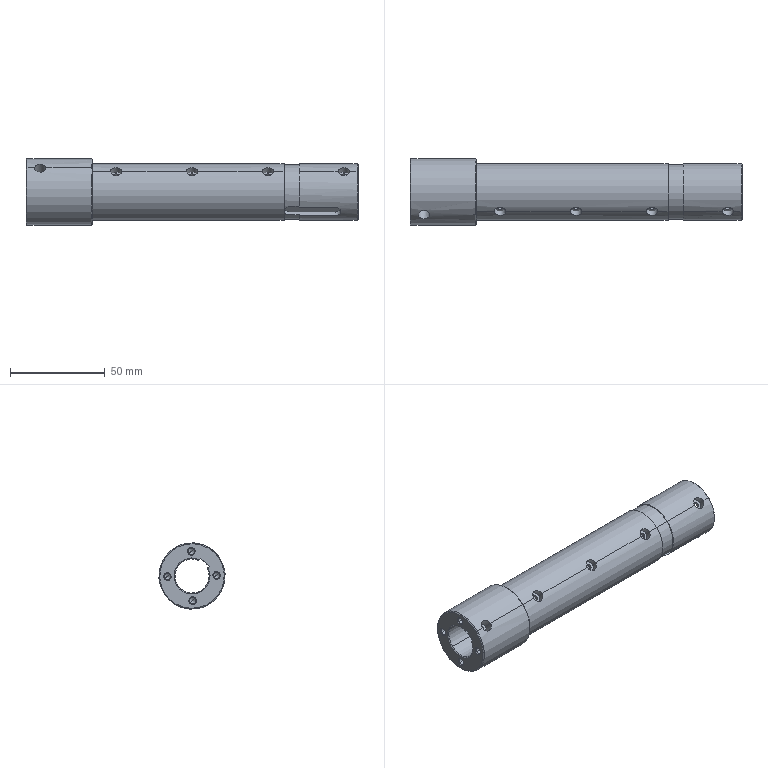Component | SolidWorks | JJDJR-3060-E-002-1 | 1 solid | 112 faces | box 175 x 35 x 35 mm | volume 83191 mm3 | cylinder 53 | cone 41 | plane 18 | commonest cylinder face diameters 6 x12 3.4 x10 2.5 x8 3.3 x8 30 x4 18 x4 29 x3 19 x2 | material 40Cr
build123d program:
from build123d import *

# Parameters (mm, degrees)
CHAMFER2_SIZE                                   = 0.5
M4_TAPPED_HOLE1_D                               = 3.3
M4_TAPPED_HOLE1_DEPTH                           = 14.1
M4_TAPPED_HOLE1_CSINK_D                         = 4.05
M4_TAPPED_HOLE1_CSINK_ANGLE                     = 90
M4_TAPPED_HOLE1_TIP                             = 0.9914
M3_TAPPED_HOLE1_D                               = 2.5
M3_TAPPED_HOLE1_DEPTH                           = 11.5
M3_TAPPED_HOLE1_CSINK_D                         = 3.05
M3_TAPPED_HOLE1_CSINK_ANGLE                     = 90
M3_TAPPED_HOLE1_TIP                             = 0.7511
CUT_EXTRUDE2_START                              = 12
CUT_EXTRUDE2_DEPTH                              = 10
SKETCH11_R                                      = 9
CUT_EXTRUDE3_DEPTH                              = 177.741
SKETCH13_W                                      = 8
SKETCH13_H                                      = 0.5
CHAMFER5_SIZE                                   = 0.5
CHAMFER6_SIZE                                   = 0.5
SKETCH15_W                                      = 55
SKETCH15_H                                      = 9.5
SKETCH16_W                                      = 6
SKETCH16_H                                      = 6
CUT_EXTRUDE5_DEPTH                              = 177.741
M3_HEX_SOCKET_HEAD_CAP_SCREW_CBORE1_D           = 3.4
M3_HEX_SOCKET_HEAD_CAP_SCREW_CBORE1_DEPTH       = 15
M3_HEX_SOCKET_HEAD_CAP_SCREW_CBORE1_CBORE_D     = 6
M3_HEX_SOCKET_HEAD_CAP_SCREW_CBORE1_CBORE_DEPTH = 6
M3_HEX_SOCKET_HEAD_CAP_SCREW_CBORE1_TIP         = 1.021


with BuildPart() as part:
    # Sketch1 → Revolve1 (revolve)
    with BuildSketch(Plane.XY, mode=Mode.PRIVATE) as revolve1_sk:
        Polygon((35, 17.5), (35, 15), (175, 15), (175, 6), (0, 6), (0, 17.5), align=None)
    revolve(revolve1_sk.sketch.rotate(Axis((0, 0, 0), (1, 0, 0)), 90), axis=Axis((0, 0, 0), (1, 0, 0)))

    # Chamfer2
    chamfer2_edges = [part.edges().sort_by_distance(p)[0] for p in [
        (0, 0, -17.5),
        (175, 0, -15),
        (35, 0, -17.5),
    ]]
    chamfer(chamfer2_edges, length=CHAMFER2_SIZE)

    # M4 Tapped Hole1
    with Locations(Plane.ZY):
        with Locations((-9.192, -9.192), (9.192, 9.192), (-9.192, 9.192), (9.192, -9.192)):
            CounterSinkHole(M4_TAPPED_HOLE1_D / 2, M4_TAPPED_HOLE1_CSINK_D / 2, depth=M4_TAPPED_HOLE1_DEPTH, counter_sink_angle=M4_TAPPED_HOLE1_CSINK_ANGLE)
            with Locations((0, 0, -(M4_TAPPED_HOLE1_DEPTH + M4_TAPPED_HOLE1_TIP / 2))):  # 118° drill point
                Cone(0, M4_TAPPED_HOLE1_D / 2, M4_TAPPED_HOLE1_TIP, mode=Mode.SUBTRACT)

    # M3 Tapped Hole1
    with Locations(Plane(origin=(175, 0, 0), x_dir=(0, 0, -1), z_dir=(1, 0, 0))):
        with Locations((8.485, -8.485), (8.485, 8.485), (-8.485, 8.485), (-8.485, -8.485)):
            CounterSinkHole(M3_TAPPED_HOLE1_D / 2, M3_TAPPED_HOLE1_CSINK_D / 2, depth=M3_TAPPED_HOLE1_DEPTH, counter_sink_angle=M3_TAPPED_HOLE1_CSINK_ANGLE)
            with Locations((0, 0, -(M3_TAPPED_HOLE1_DEPTH + M3_TAPPED_HOLE1_TIP / 2))):  # 118° drill point
                Cone(0, M3_TAPPED_HOLE1_D / 2, M3_TAPPED_HOLE1_TIP, mode=Mode.SUBTRACT)

    # Sketch7 → Cut-Extrude2 (cut)
    with BuildSketch(Plane(origin=(0, 0, 0), x_dir=(1, 0, 0), z_dir=(0, 1, 0)).offset(CUT_EXTRUDE2_START)):
        with BuildLine():
            Line((163, -3), (139, -3))
            ThreePointArc((139, -3), (136, 0), (139, 3))
            Line((139, 3), (163, 3))
            ThreePointArc((163, 3), (166, 0), (163, -3))
        make_face()
    extrude(amount=CUT_EXTRUDE2_DEPTH, mode=Mode.SUBTRACT)

    # Sketch11 → Cut-Extrude3 (cut, through all)
    with BuildSketch(Plane.ZY):
        Circle(SKETCH11_R)
    extrude(amount=-CUT_EXTRUDE3_DEPTH, mode=Mode.SUBTRACT)

    # Sketch13 → Cut-Revolve1 (revolve, cut)
    with BuildSketch(Plane(origin=(0, 0, 0), x_dir=(1, 0, 0), z_dir=(0, 1, 0)), mode=Mode.PRIVATE) as cut_revolve1_sk:
        with Locations((140, 14.75)):
            Rectangle(SKETCH13_W, SKETCH13_H)
    revolve(cut_revolve1_sk.sketch.rotate(Axis((0, 0, 0), (1, 0, 0)), 180), axis=Axis((0, 0, 0), (1, 0, 0)), mode=Mode.SUBTRACT)

    # Chamfer5
    chamfer5_edges = [part.edges().sort_by_distance(p)[0] for p in [
        (0, 0, -9),
    ]]
    chamfer(chamfer5_edges, length=CHAMFER5_SIZE)

    # Chamfer6
    chamfer6_edges = [part.edges().sort_by_distance(p)[0] for p in [
        (175, 0, -9),
    ]]
    chamfer(chamfer6_edges, length=CHAMFER6_SIZE)

    # Sketch15 → Cut-Revolve2 (revolve, cut)
    with BuildSketch(Plane(origin=(0, 0, 0), x_dir=(1, 0, 0), z_dir=(0, 1, 0))):
        with Locations((87.5, 4.75)):
            Rectangle(SKETCH15_W, SKETCH15_H)
    revolve(axis=Axis((0, 0, 0), (1, 0, 0)), mode=Mode.SUBTRACT)

    # Sketch16 → Cut-Extrude5 (cut, through all)
    with BuildSketch(Plane(origin=(175, 0, 0), x_dir=(0, 0, -1), z_dir=(1, 0, 0))):
        with Locations((7, 0)):
            Rectangle(SKETCH16_W, SKETCH16_H)
    extrude(amount=-CUT_EXTRUDE5_DEPTH, mode=Mode.SUBTRACT)

    # M3 Hex Socket Head Cap Screw CBORE1
    with Locations(Plane(origin=(0, 0, -17.5), x_dir=(-1, 0, 0), z_dir=(0, 0, -1))):
        with Locations((-7.5, 0), (-87.5, 0), (-127.5, 0), (-167.5, 0), (-47.5, 0)):
            CounterBoreHole(M3_HEX_SOCKET_HEAD_CAP_SCREW_CBORE1_D / 2, M3_HEX_SOCKET_HEAD_CAP_SCREW_CBORE1_CBORE_D / 2, M3_HEX_SOCKET_HEAD_CAP_SCREW_CBORE1_CBORE_DEPTH, depth=M3_HEX_SOCKET_HEAD_CAP_SCREW_CBORE1_DEPTH)
            with Locations((0, 0, -(M3_HEX_SOCKET_HEAD_CAP_SCREW_CBORE1_DEPTH + M3_HEX_SOCKET_HEAD_CAP_SCREW_CBORE1_TIP / 2))):  # 118° drill point
                Cone(0, M3_HEX_SOCKET_HEAD_CAP_SCREW_CBORE1_D / 2, M3_HEX_SOCKET_HEAD_CAP_SCREW_CBORE1_TIP, mode=Mode.SUBTRACT)


solid = part.part

# Placed as in the assembly
solid = solid.moved(Location((-140.59, -29.263, -16.52), (-136.43, 0, 0)))